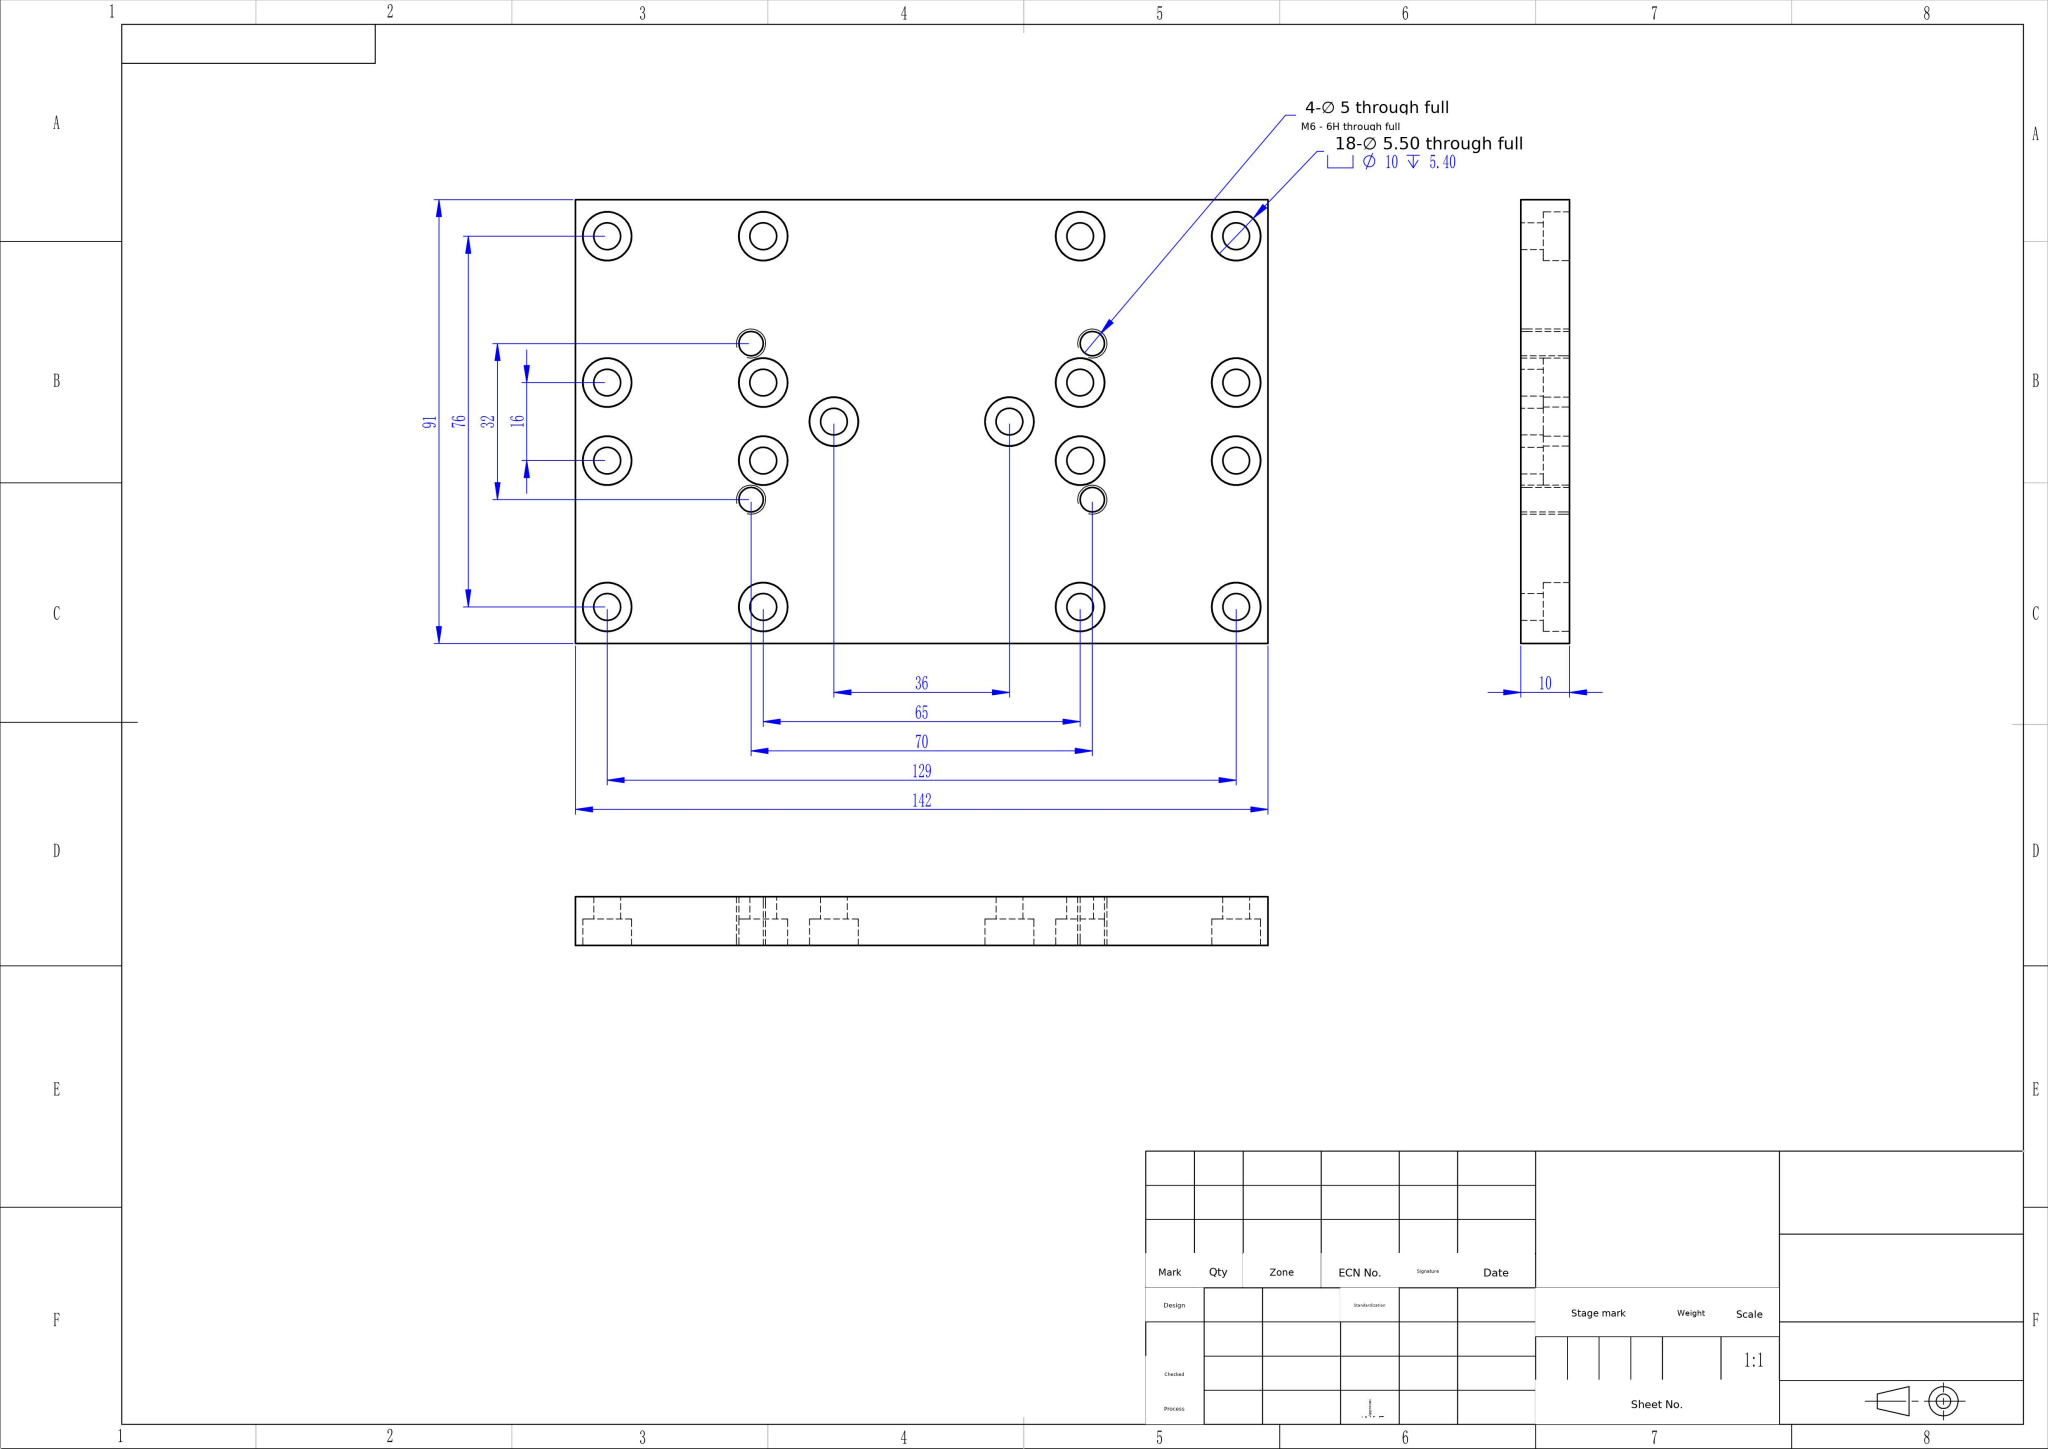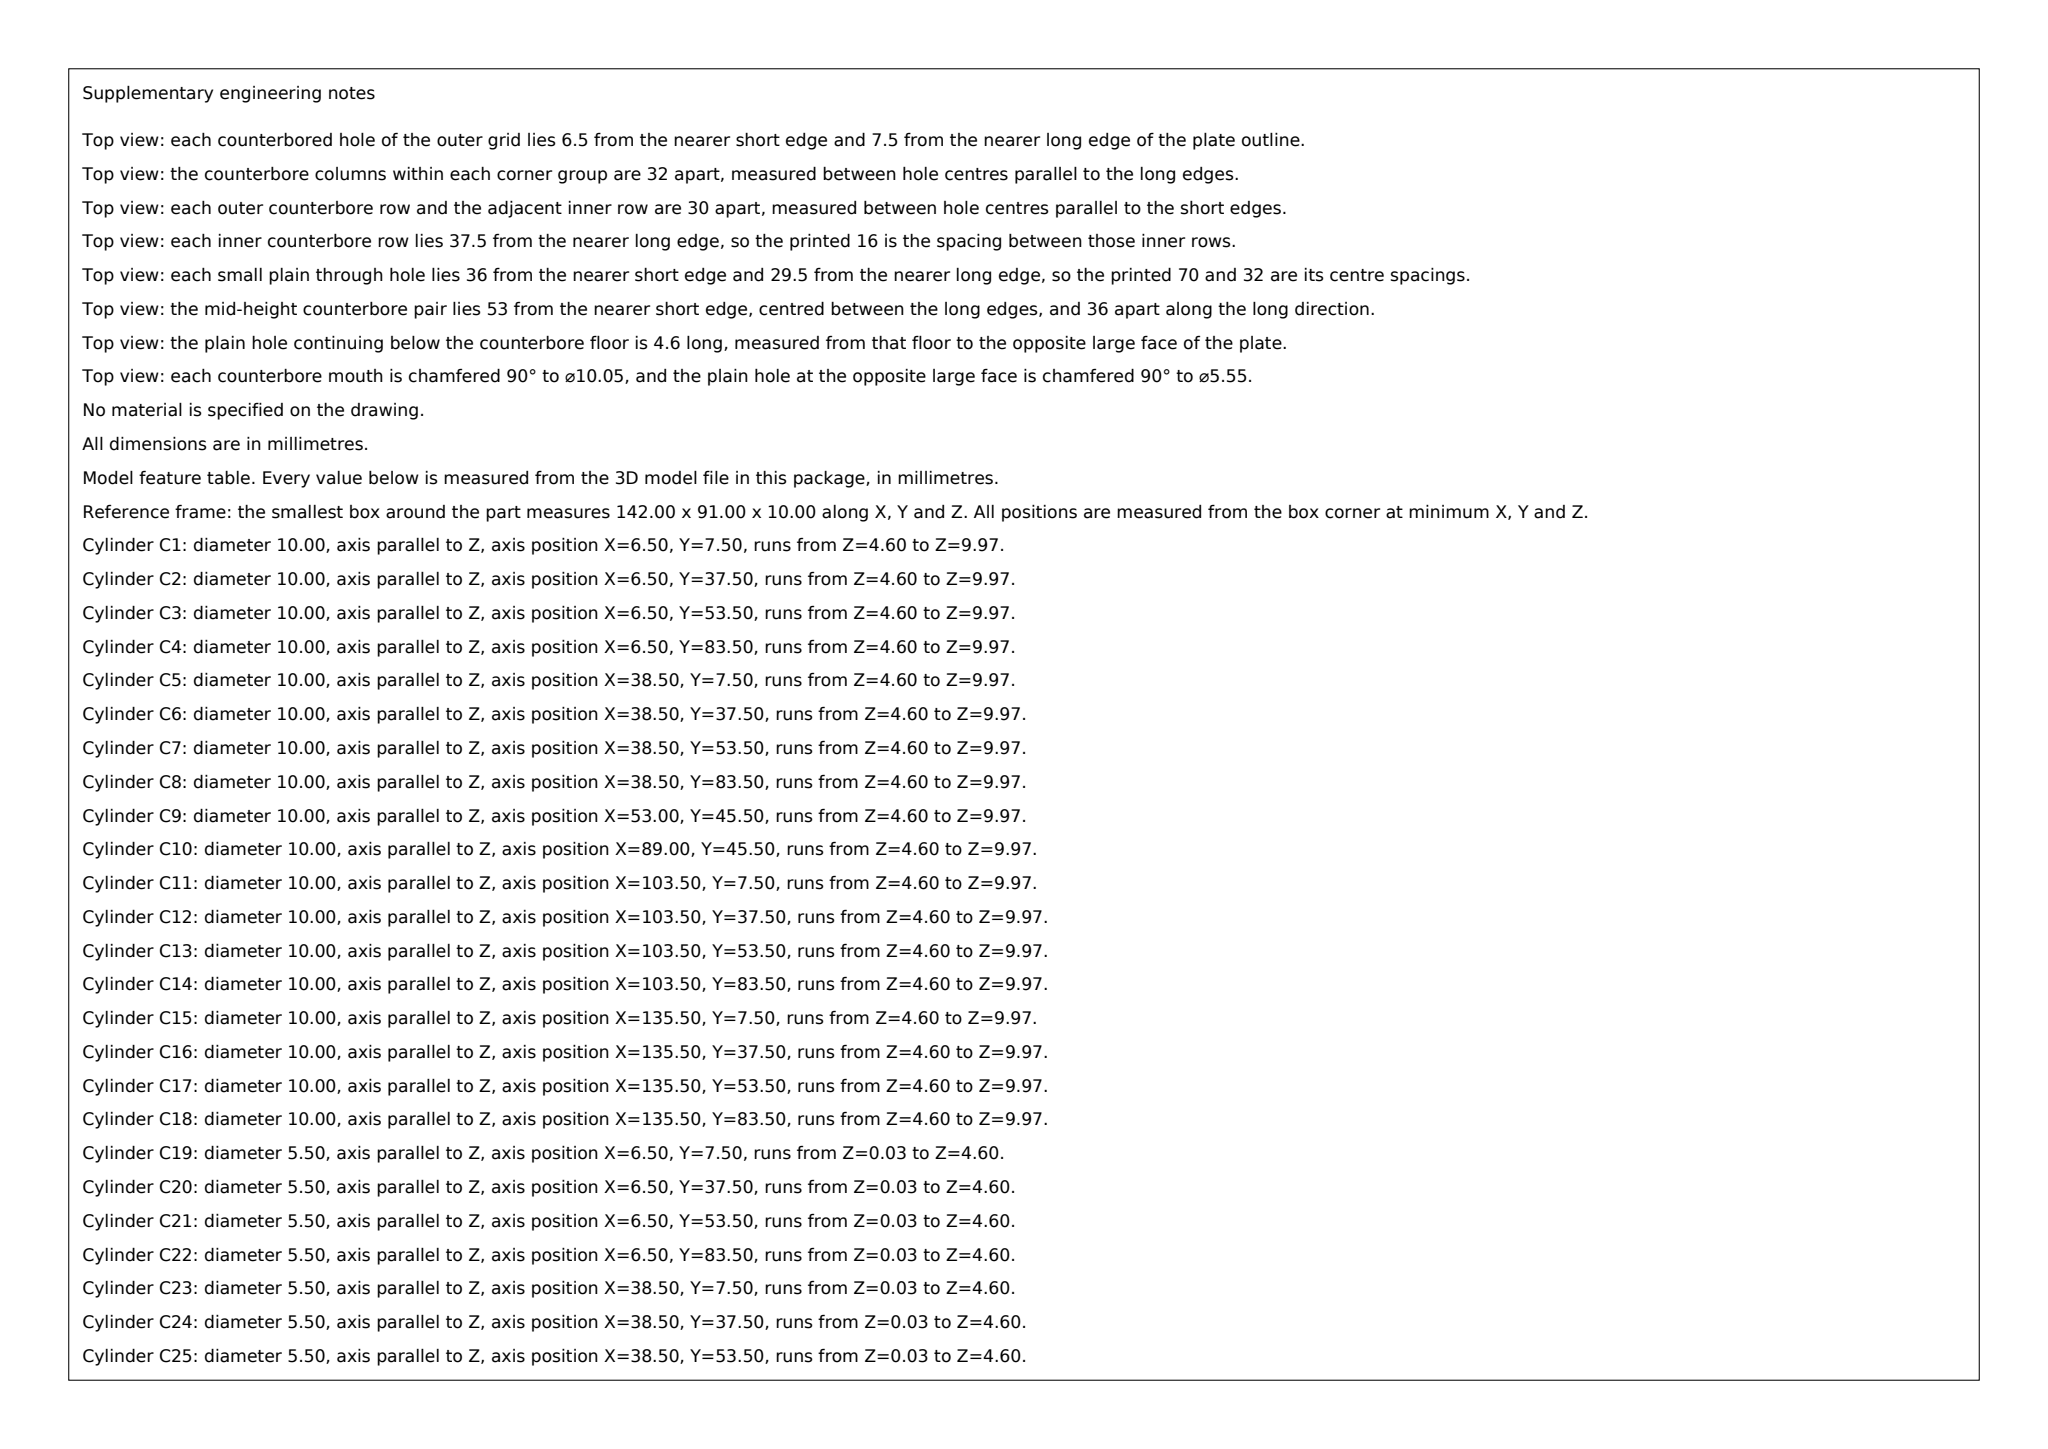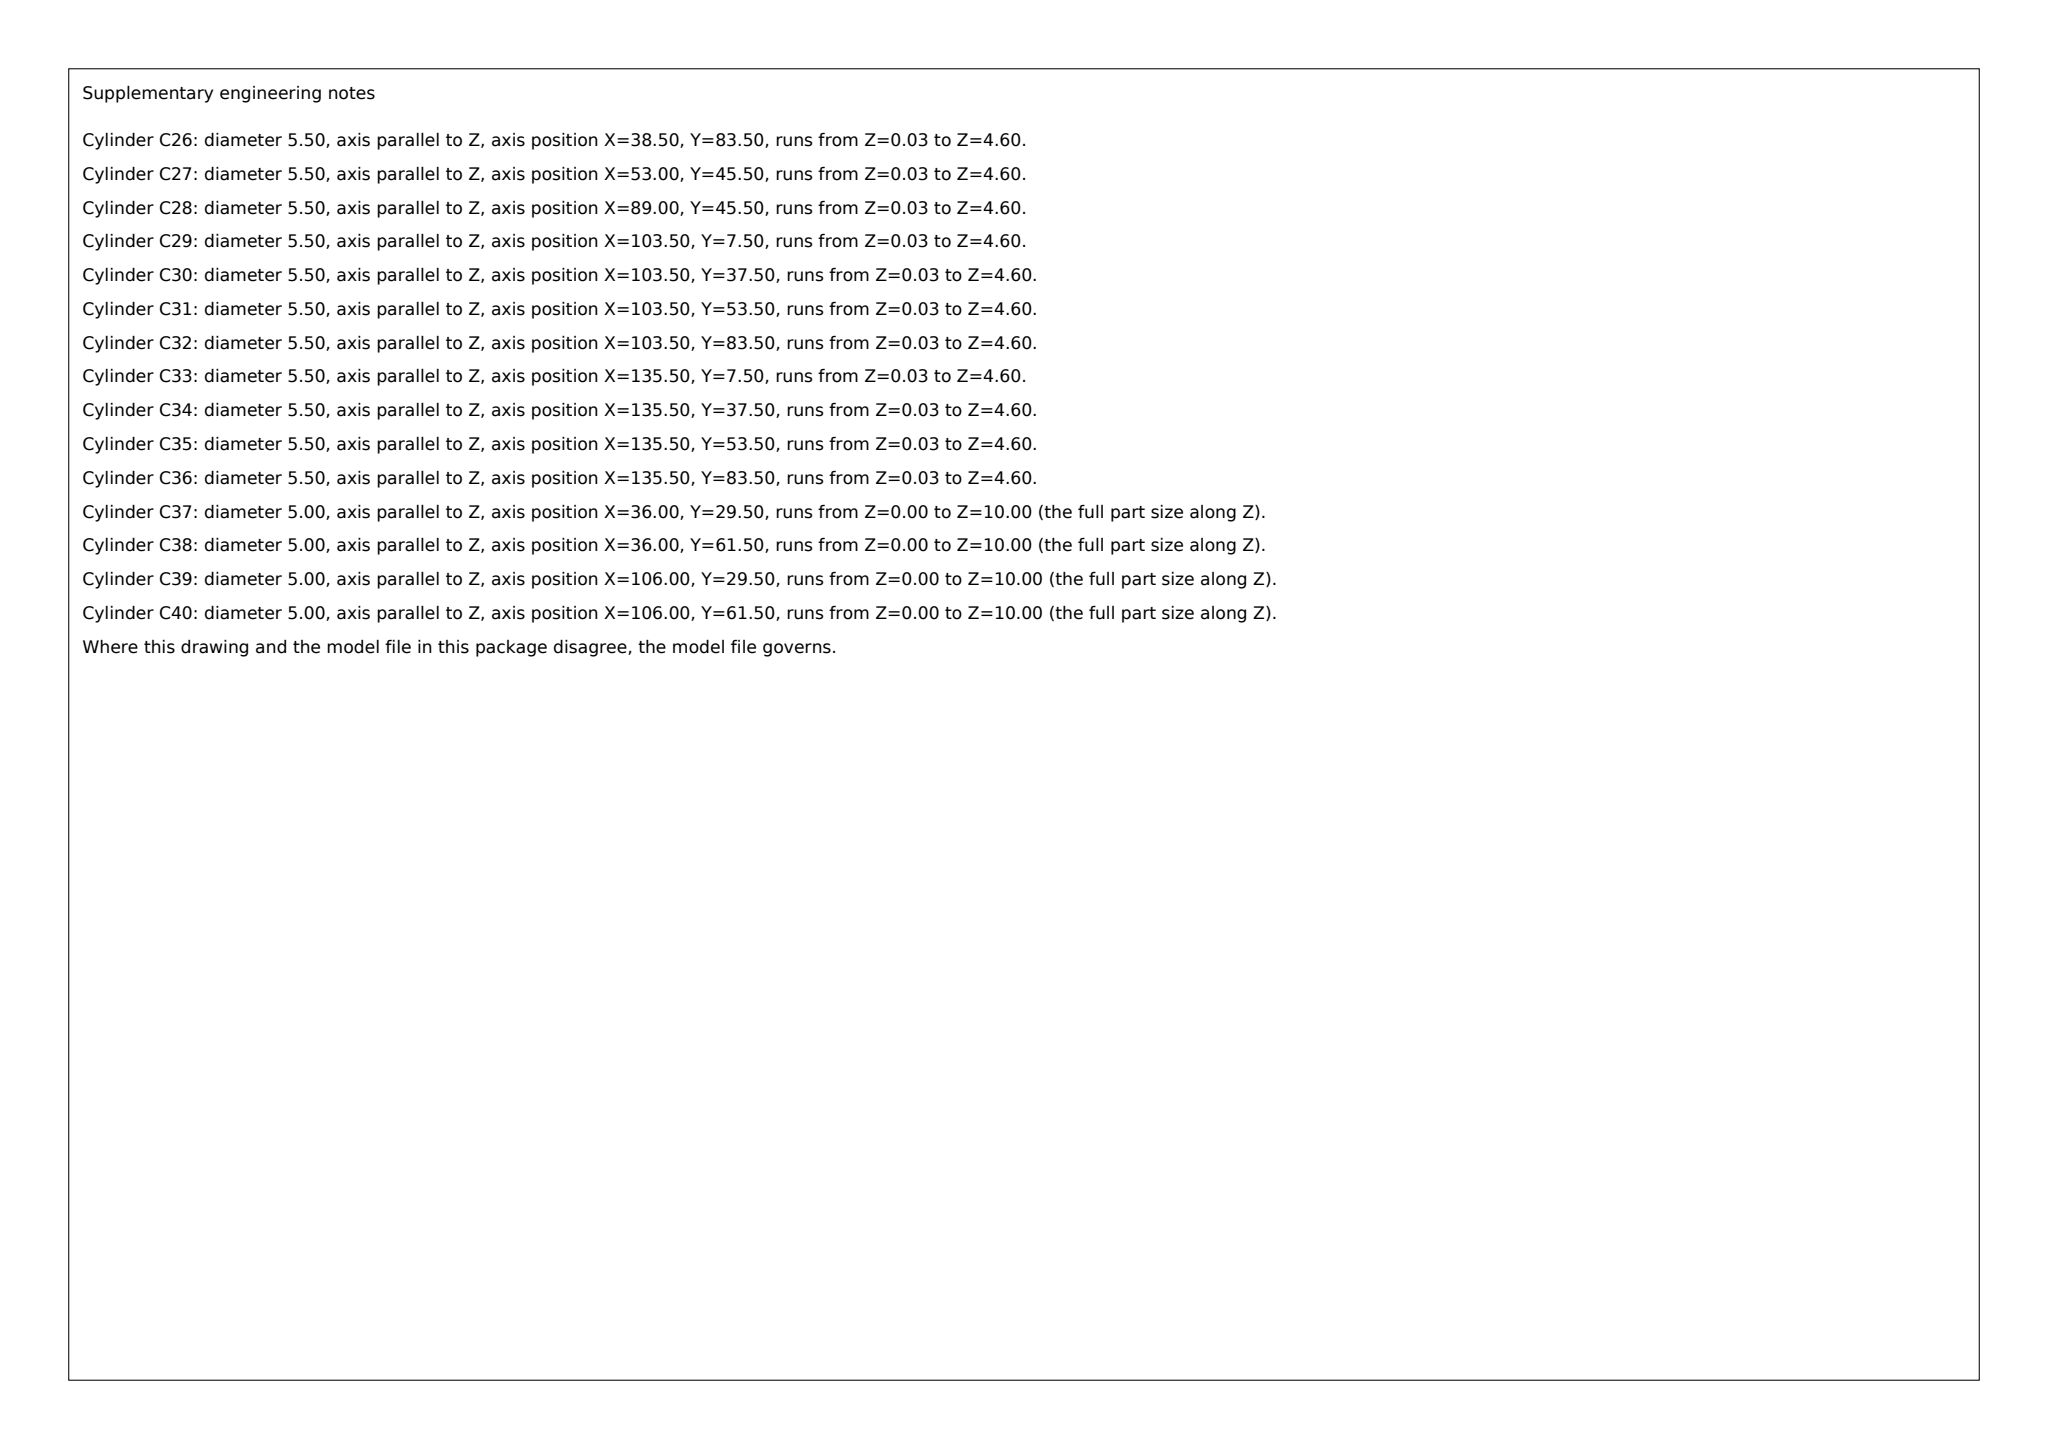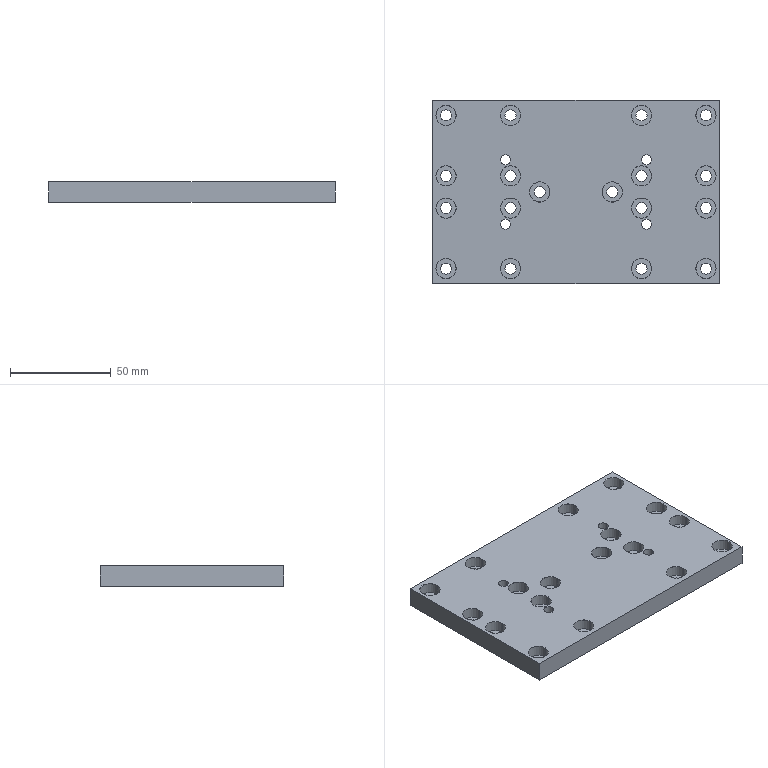Part | SolidWorks | mm | 1 solid | 176 faces | box 142 x 91 x 10 mm | volume 118833 mm3 | cylinder 80 | cone 72 | plane 24 | commonest cylinder face diameters 10 x36 5.5 x36 5 x8
Drawing notes:
18X Ø5.5 THRU, C'BORE Ø10 DP 5.40 FROM TOP FACE (Z=10); C'BORE CENTERS AT X=6.5, 38.5, 103.5, 135.5 WITH Y=7.5, 37.5, 53.5, 83.5 PLUS X=53.0 AND X=89.0 AT Y=45.5, FROM LOWER-LEFT CORNER | from the solid: cylinders: 18X Ø5.5 z-axis from 0.0 to 4.6 and 18X Ø10.0 z-axis from 4.6 to 10.0 at the listed x,y positions
BREAK EDGE AT MOUTH OF EACH Ø10 COUNTERBORE: 90° CHAMFER TO Ø10.05 ON TOP FACE (Z=10) | from the solid: cones: included_angle 90.0, ref_dia 10.05, bbox_from z=10.0 at counterbore locations
build123d program:
from build123d import *

# Parameters (mm, degrees)
SKIZZE1_W                                     = 142
SKIZZE1_H                                     = 91
AUFSATZ_LINEAR_AUSTRAGEN1_DEPTH               = 10
SKIZZE3_R                                     = 2.5
SCHNITT_LINEAR_AUSTRAGEN2_DEPTH               = 10
SKIZZE4_R                                     = 2.5
SCHNITT_LINEAR_AUSTRAGEN3_DEPTH               = 10
M6_GEWINDEBOHRUNG1_D                          = 5
STIRNSENKUNG_F_R_M5_ZYLINDERSCHRAUBE_2_COUNT  = 2
STIRNSENKUNG_F_R_M5_ZYLINDERSCHRAUBE_2_PITCH  = 32
STIRNSENKUNG_F_R_M5_ZYLINDERSCHRAUBE_3_COUNT  = 2
STIRNSENKUNG_F_R_M5_ZYLINDERSCHRAUBE_3_PITCH  = 30
STIRNSENKUNG_F_R_M5_ZYLINDERSCHRAUBE_4_COUNT  = 2
STIRNSENKUNG_F_R_M5_ZYLINDERSCHRAUBE_4_PITCH  = 43.863
STIRNSENKUNG_F_R_M5_ZYLINDERSCHRAUBE_5_COUNT  = 2
STIRNSENKUNG_F_R_M5_ZYLINDERSCHRAUBE_5_PITCH  = 60.052
STIRNSENKUNG_F_R_M5_ZYLINDERSCHRAUBE_6_COUNT  = 2
STIRNSENKUNG_F_R_M5_ZYLINDERSCHRAUBE_6_PITCH  = 90.831
STIRNSENKUNG_F_R_M5_ZYLINDERSCHRAUBE_7_COUNT  = 2
STIRNSENKUNG_F_R_M5_ZYLINDERSCHRAUBE_7_PITCH  = 46
STIRNSENKUNG_F_R_M5_ZYLINDERSCHRAUBE_8_COUNT  = 2
STIRNSENKUNG_F_R_M5_ZYLINDERSCHRAUBE_8_PITCH  = 76
STIRNSENKUNG_F_R_M5_ZYLINDERSCHRAUBE_9_COUNT  = 2
STIRNSENKUNG_F_R_M5_ZYLINDERSCHRAUBE_9_PITCH  = 82.462
STIRNSENKUNG_F_R_M5_ZYLINDERSCHRAUBE_10_COUNT = 2
STIRNSENKUNG_F_R_M5_ZYLINDERSCHRAUBE_10_PITCH = 123.227
STIRNSENKUNG_F_R_M5_ZYLINDERSCHRAUBE_11_COUNT = 2
STIRNSENKUNG_F_R_M5_ZYLINDERSCHRAUBE_11_PITCH = 149.723
STIRNSENKUNG_F_R_M5_ZYLINDERSCHRAUBE_12_COUNT = 2
STIRNSENKUNG_F_R_M5_ZYLINDERSCHRAUBE_12_PITCH = 107.355
STIRNSENKUNG_F_R_M5_ZYLINDERSCHRAUBE_13_COUNT = 2
STIRNSENKUNG_F_R_M5_ZYLINDERSCHRAUBE_13_PITCH = 101.533
STIRNSENKUNG_F_R_M5_ZYLINDERSCHRAUBE_14_COUNT = 2
STIRNSENKUNG_F_R_M5_ZYLINDERSCHRAUBE_14_PITCH = 132.442
STIRNSENKUNG_F_R_M5_ZYLINDERSCHRAUBE_15_COUNT = 2
STIRNSENKUNG_F_R_M5_ZYLINDERSCHRAUBE_15_PITCH = 136.956
STIRNSENKUNG_F_R_M5_ZYLINDERSCHRAUBE_16_COUNT = 2
STIRNSENKUNG_F_R_M5_ZYLINDERSCHRAUBE_16_PITCH = 129
STIRNSENKUNG_F_R_M5_ZYLINDERSCHRAUBE_17_COUNT = 2
STIRNSENKUNG_F_R_M5_ZYLINDERSCHRAUBE_17_PITCH = 97
STIRNSENKUNG_F_R_M5_ZYLINDERSCHRAUBE_18_COUNT = 2
STIRNSENKUNG_F_R_M5_ZYLINDERSCHRAUBE_18_PITCH = 56.036


with BuildPart() as part:
    # Skizze1 → Aufsatz-Linear austragen1 (new body)
    with BuildSketch(Plane.XY):
        with Locations((-71, 45.5)):
            Rectangle(SKIZZE1_W, SKIZZE1_H)
    extrude(amount=AUFSATZ_LINEAR_AUSTRAGEN1_DEPTH)

    # Skizze3 → Schnitt-Linear austragen2 (cut)
    with BuildSketch(Plane.XY.offset(10)):
        with Locations((-135.5, 83.5)):
            Circle(SKIZZE3_R)
        with Locations((-103.5, 83.5)):
            Circle(SKIZZE3_R)
        with Locations((-135.5, 37.5)):
            Circle(SKIZZE3_R)
        with Locations((-103.5, 37.5)):
            Circle(SKIZZE3_R)
        with Locations((-38.5, 83.5)):
            Circle(SKIZZE3_R)
        with Locations((-38.5, 53.5)):
            Circle(SKIZZE3_R)
        with Locations((-6.5, 53.5)):
            Circle(SKIZZE3_R)
        with Locations((-6.5, 83.5)):
            Circle(SKIZZE3_R)
        with Locations((-38.5, 37.5)):
            Circle(SKIZZE3_R)
        with Locations((-6.5, 37.5)):
            Circle(SKIZZE3_R)
        with Locations((-38.5, 7.5)):
            Circle(SKIZZE3_R)
        with Locations((-6.5, 7.5)):
            Circle(SKIZZE3_R)
        with Locations((-103.5, 7.5)):
            Circle(SKIZZE3_R)
        with Locations((-135.5, 7.5)):
            Circle(SKIZZE3_R)
        with Locations((-135.5, 53.5)):
            Circle(SKIZZE3_R)
        with Locations((-103.5, 53.5)):
            Circle(SKIZZE3_R)
    extrude(amount=-SCHNITT_LINEAR_AUSTRAGEN2_DEPTH, mode=Mode.SUBTRACT)

    # Skizze4 → Schnitt-Linear austragen3 (cut)
    with BuildSketch(Plane.XY.offset(10)):
        with Locations((-89, 45.5)):
            Circle(SKIZZE4_R)
        with Locations((-53, 45.5)):
            Circle(SKIZZE4_R)
    extrude(amount=-SCHNITT_LINEAR_AUSTRAGEN3_DEPTH, mode=Mode.SUBTRACT)

    # M6 Gewindebohrung1 (through all)
    with Locations(Plane(origin=(-106, 61.5, 10), x_dir=(1, 0, 0), z_dir=(0, 0, 1))):
        with Locations((0, 0), (70, 0), (70, -32), (0, -32)):
            Hole(M6_GEWINDEBOHRUNG1_D / 2)

    # Skizze6 → Stirnsenkung f_r M5 Zylinderschraube mit (revolve, cut)
    with BuildSketch(Plane(origin=(-135.5, 83.5, 10), x_dir=(0, -1, 0), z_dir=(1, 0, 0))):
        Polygon((0, 0), (0, 10), (2.775, 10), (2.75, 9.975), (2.75, 5.4), (5, 5.4), (5, 0.025), (5.025, 0), align=None)
    stirnsenkung_f_r_m5_zylinderschraube_mit = revolve(axis=Axis((-135.5, 83.5, 16.35), (0, 0, -1)), mode=Mode.SUBTRACT)

    # Stirnsenkung f_r M5 Zylinderschraube 2: Stirnsenkung f_r M5 Zylinderschraube mit ×2
    with Locations(*[(i * STIRNSENKUNG_F_R_M5_ZYLINDERSCHRAUBE_2_PITCH, 0, 0) for i in range(1, STIRNSENKUNG_F_R_M5_ZYLINDERSCHRAUBE_2_COUNT)]):
        add(stirnsenkung_f_r_m5_zylinderschraube_mit, mode=Mode.SUBTRACT)

    # Stirnsenkung f_r M5 Zylinderschraube 3: Stirnsenkung f_r M5 Zylinderschraube mit ×2
    with Locations(*[(0, -i * STIRNSENKUNG_F_R_M5_ZYLINDERSCHRAUBE_3_PITCH, 0) for i in range(1, STIRNSENKUNG_F_R_M5_ZYLINDERSCHRAUBE_3_COUNT)]):
        add(stirnsenkung_f_r_m5_zylinderschraube_mit, mode=Mode.SUBTRACT)

    # Stirnsenkung f_r M5 Zylinderschraube 4: Stirnsenkung f_r M5 Zylinderschraube mit ×2
    with Locations(*[Vector(0.7295, -0.6839, 0) * (i * STIRNSENKUNG_F_R_M5_ZYLINDERSCHRAUBE_4_PITCH) for i in range(1, STIRNSENKUNG_F_R_M5_ZYLINDERSCHRAUBE_4_COUNT)]):
        add(stirnsenkung_f_r_m5_zylinderschraube_mit, mode=Mode.SUBTRACT)

    # Stirnsenkung f_r M5 Zylinderschraube 5: Stirnsenkung f_r M5 Zylinderschraube mit ×2
    with Locations(*[Vector(0.7743, -0.6328, 0) * (i * STIRNSENKUNG_F_R_M5_ZYLINDERSCHRAUBE_5_PITCH) for i in range(1, STIRNSENKUNG_F_R_M5_ZYLINDERSCHRAUBE_5_COUNT)]):
        add(stirnsenkung_f_r_m5_zylinderschraube_mit, mode=Mode.SUBTRACT)

    # Stirnsenkung f_r M5 Zylinderschraube 6: Stirnsenkung f_r M5 Zylinderschraube mit ×2
    with Locations(*[Vector(0.9083, -0.4184, 0) * (i * STIRNSENKUNG_F_R_M5_ZYLINDERSCHRAUBE_6_PITCH) for i in range(1, STIRNSENKUNG_F_R_M5_ZYLINDERSCHRAUBE_6_COUNT)]):
        add(stirnsenkung_f_r_m5_zylinderschraube_mit, mode=Mode.SUBTRACT)

    # Stirnsenkung f_r M5 Zylinderschraube 7: Stirnsenkung f_r M5 Zylinderschraube mit ×2
    with Locations(*[(0, -i * STIRNSENKUNG_F_R_M5_ZYLINDERSCHRAUBE_7_PITCH, 0) for i in range(1, STIRNSENKUNG_F_R_M5_ZYLINDERSCHRAUBE_7_COUNT)]):
        add(stirnsenkung_f_r_m5_zylinderschraube_mit, mode=Mode.SUBTRACT)

    # Stirnsenkung f_r M5 Zylinderschraube 8: Stirnsenkung f_r M5 Zylinderschraube mit ×2
    with Locations(*[(0, -i * STIRNSENKUNG_F_R_M5_ZYLINDERSCHRAUBE_8_PITCH, 0) for i in range(1, STIRNSENKUNG_F_R_M5_ZYLINDERSCHRAUBE_8_COUNT)]):
        add(stirnsenkung_f_r_m5_zylinderschraube_mit, mode=Mode.SUBTRACT)

    # Stirnsenkung f_r M5 Zylinderschraube 9: Stirnsenkung f_r M5 Zylinderschraube mit ×2
    with Locations(*[Vector(0.3881, -0.9216, 0) * (i * STIRNSENKUNG_F_R_M5_ZYLINDERSCHRAUBE_9_PITCH) for i in range(1, STIRNSENKUNG_F_R_M5_ZYLINDERSCHRAUBE_9_COUNT)]):
        add(stirnsenkung_f_r_m5_zylinderschraube_mit, mode=Mode.SUBTRACT)

    # Stirnsenkung f_r M5 Zylinderschraube 10: Stirnsenkung f_r M5 Zylinderschraube mit ×2
    with Locations(*[Vector(0.7872, -0.6167, 0) * (i * STIRNSENKUNG_F_R_M5_ZYLINDERSCHRAUBE_10_PITCH) for i in range(1, STIRNSENKUNG_F_R_M5_ZYLINDERSCHRAUBE_10_COUNT)]):
        add(stirnsenkung_f_r_m5_zylinderschraube_mit, mode=Mode.SUBTRACT)

    # Stirnsenkung f_r M5 Zylinderschraube 11: Stirnsenkung f_r M5 Zylinderschraube mit ×2
    with Locations(*[Vector(0.8616, -0.5076, 0) * (i * STIRNSENKUNG_F_R_M5_ZYLINDERSCHRAUBE_11_PITCH) for i in range(1, STIRNSENKUNG_F_R_M5_ZYLINDERSCHRAUBE_11_COUNT)]):
        add(stirnsenkung_f_r_m5_zylinderschraube_mit, mode=Mode.SUBTRACT)

    # Stirnsenkung f_r M5 Zylinderschraube 12: Stirnsenkung f_r M5 Zylinderschraube mit ×2
    with Locations(*[Vector(0.9035, -0.4285, 0) * (i * STIRNSENKUNG_F_R_M5_ZYLINDERSCHRAUBE_12_PITCH) for i in range(1, STIRNSENKUNG_F_R_M5_ZYLINDERSCHRAUBE_12_COUNT)]):
        add(stirnsenkung_f_r_m5_zylinderschraube_mit, mode=Mode.SUBTRACT)

    # Stirnsenkung f_r M5 Zylinderschraube 13: Stirnsenkung f_r M5 Zylinderschraube mit ×2
    with Locations(*[Vector(0.9554, -0.2955, 0) * (i * STIRNSENKUNG_F_R_M5_ZYLINDERSCHRAUBE_13_PITCH) for i in range(1, STIRNSENKUNG_F_R_M5_ZYLINDERSCHRAUBE_13_COUNT)]):
        add(stirnsenkung_f_r_m5_zylinderschraube_mit, mode=Mode.SUBTRACT)

    # Stirnsenkung f_r M5 Zylinderschraube 14: Stirnsenkung f_r M5 Zylinderschraube mit ×2
    with Locations(*[Vector(0.974, -0.2265, 0) * (i * STIRNSENKUNG_F_R_M5_ZYLINDERSCHRAUBE_14_PITCH) for i in range(1, STIRNSENKUNG_F_R_M5_ZYLINDERSCHRAUBE_14_COUNT)]):
        add(stirnsenkung_f_r_m5_zylinderschraube_mit, mode=Mode.SUBTRACT)

    # Stirnsenkung f_r M5 Zylinderschraube 15: Stirnsenkung f_r M5 Zylinderschraube mit ×2
    with Locations(*[Vector(0.9419, -0.3359, 0) * (i * STIRNSENKUNG_F_R_M5_ZYLINDERSCHRAUBE_15_PITCH) for i in range(1, STIRNSENKUNG_F_R_M5_ZYLINDERSCHRAUBE_15_COUNT)]):
        add(stirnsenkung_f_r_m5_zylinderschraube_mit, mode=Mode.SUBTRACT)

    # Stirnsenkung f_r M5 Zylinderschraube 16: Stirnsenkung f_r M5 Zylinderschraube mit ×2
    with Locations(*[(i * STIRNSENKUNG_F_R_M5_ZYLINDERSCHRAUBE_16_PITCH, 0, 0) for i in range(1, STIRNSENKUNG_F_R_M5_ZYLINDERSCHRAUBE_16_COUNT)]):
        add(stirnsenkung_f_r_m5_zylinderschraube_mit, mode=Mode.SUBTRACT)

    # Stirnsenkung f_r M5 Zylinderschraube 17: Stirnsenkung f_r M5 Zylinderschraube mit ×2
    with Locations(*[(i * STIRNSENKUNG_F_R_M5_ZYLINDERSCHRAUBE_17_PITCH, 0, 0) for i in range(1, STIRNSENKUNG_F_R_M5_ZYLINDERSCHRAUBE_17_COUNT)]):
        add(stirnsenkung_f_r_m5_zylinderschraube_mit, mode=Mode.SUBTRACT)

    # Stirnsenkung f_r M5 Zylinderschraube 18: Stirnsenkung f_r M5 Zylinderschraube mit ×2
    with Locations(*[Vector(0.5711, -0.8209, 0) * (i * STIRNSENKUNG_F_R_M5_ZYLINDERSCHRAUBE_18_PITCH) for i in range(1, STIRNSENKUNG_F_R_M5_ZYLINDERSCHRAUBE_18_COUNT)]):
        add(stirnsenkung_f_r_m5_zylinderschraube_mit, mode=Mode.SUBTRACT)


solid = part.part